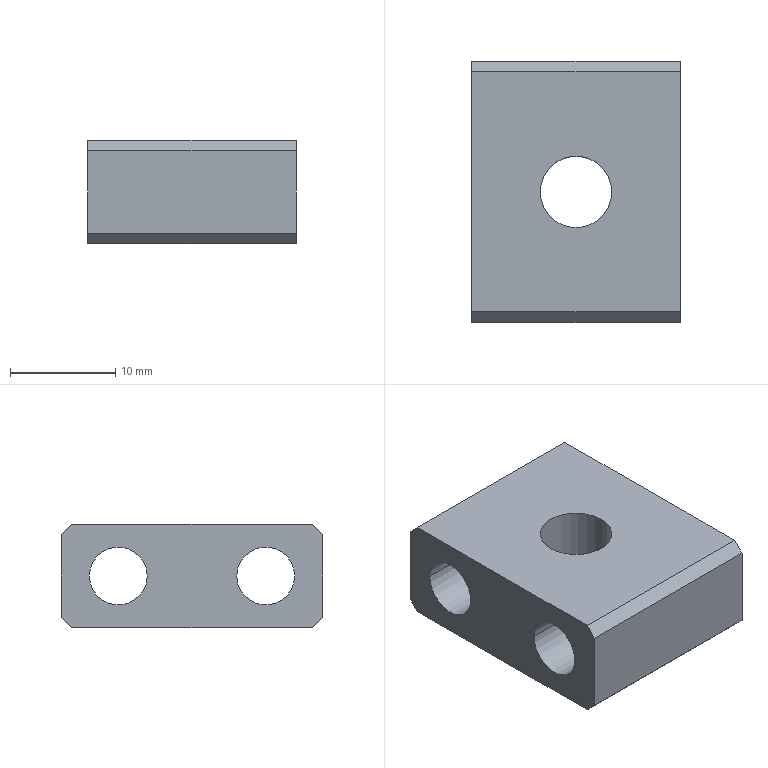Component | SolidWorks | ChainPartDrivenShaftAdjustmentBracket-4 | 1 solid | 16 faces | box 19.8 x 24.8 x 9.8 mm | volume 3476 mm3 | plane 10 | cylinder 6 | commonest cylinder face diameters 5.5 x4 6.8 x2
build123d program:
from build123d import *

# Parameters (mm, degrees)
SKETCH1_W           = 24.8
SKETCH1_H           = 9.8
SKETCH1_R           = 2.75
BOSS_EXTRUDE1_DEPTH = 9.9
M8_TAPPED_HOLE1_D   = 6.8
CHAMFER1_SIZE       = 1


with BuildPart() as part:
    # Sketch1 → Boss-Extrude1 (new, symmetric)
    with BuildSketch(Plane.XY):
        Rectangle(SKETCH1_W, SKETCH1_H)
        with Locations(Location((-7, 0, 0), (0, 0, 180))):
            Circle(SKETCH1_R, mode=Mode.SUBTRACT)
        with Locations(Location((7, 0, 0), (0, 0, 180))):
            Circle(SKETCH1_R, mode=Mode.SUBTRACT)
    extrude(amount=BOSS_EXTRUDE1_DEPTH, both=True)

    # M8 Tapped Hole1 (through all)
    with Locations(Plane(origin=(0, -4.9, 0), x_dir=(-1, 0, 0), z_dir=(0, -1, 0))):
        with Locations((0, 0)):
            Hole(M8_TAPPED_HOLE1_D / 2)

    # Chamfer1
    chamfer1_edges = [part.edges().sort_by_distance(p)[0] for p in [
        (-12.4, 4.9, 0),
        (12.4, 4.9, 0),
        (12.4, -4.9, 0),
        (-12.4, -4.9, 0),
    ]]
    chamfer(chamfer1_edges, length=CHAMFER1_SIZE)


solid = part.part

# Placed as in the assembly
solid = solid.moved(Location((70.337, -2.563, -642.304), (90, -90, 0)))